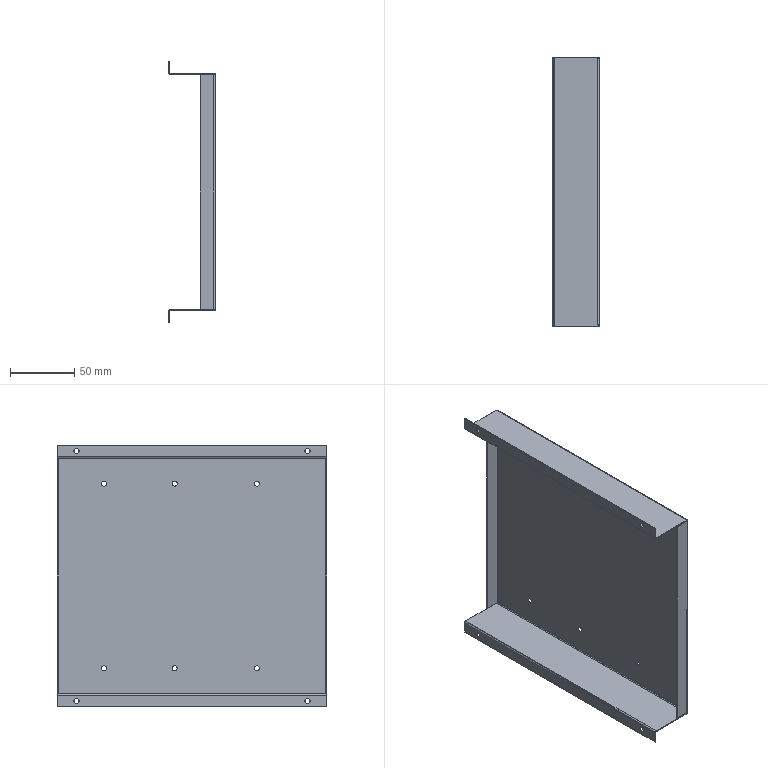Component | SolidWorks | PC-CAJ-P09-1_PM-CAJ-P52-2 | 1 solid | 78 faces | volume 42943 mm3 | plane 46 | cylinder 32 | commonest cylinder face diameters 4 x20 2.4 x6 1 x6 | material Plain Carbon Steel